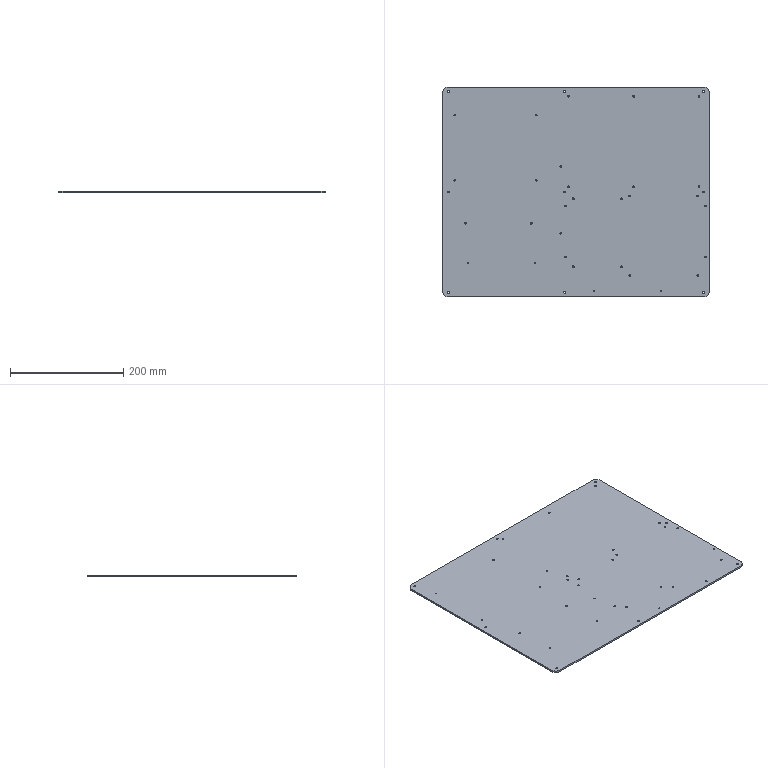CAM job | Mastercam | mm | 4 operations | part box 470 x 370 x 3
1. Contour (Ramp) | 9 - 10 平铣刀
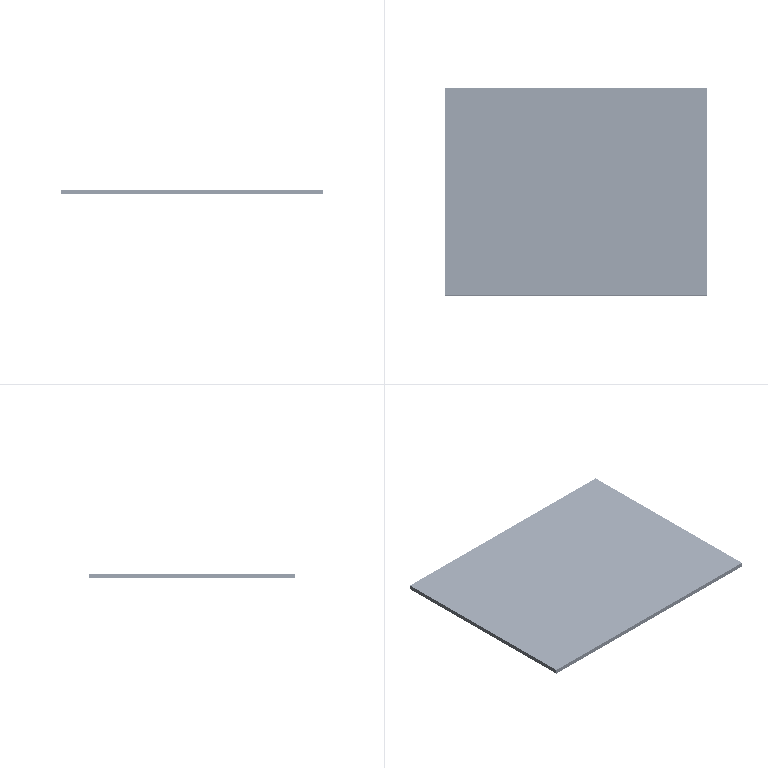2. Contour (2D) | 10 - 10 平铣刀
3. Contour (2D chamfer) | 5 - 4 倒角刀
4. Drill/Counterbore | 5 - 4 倒角刀